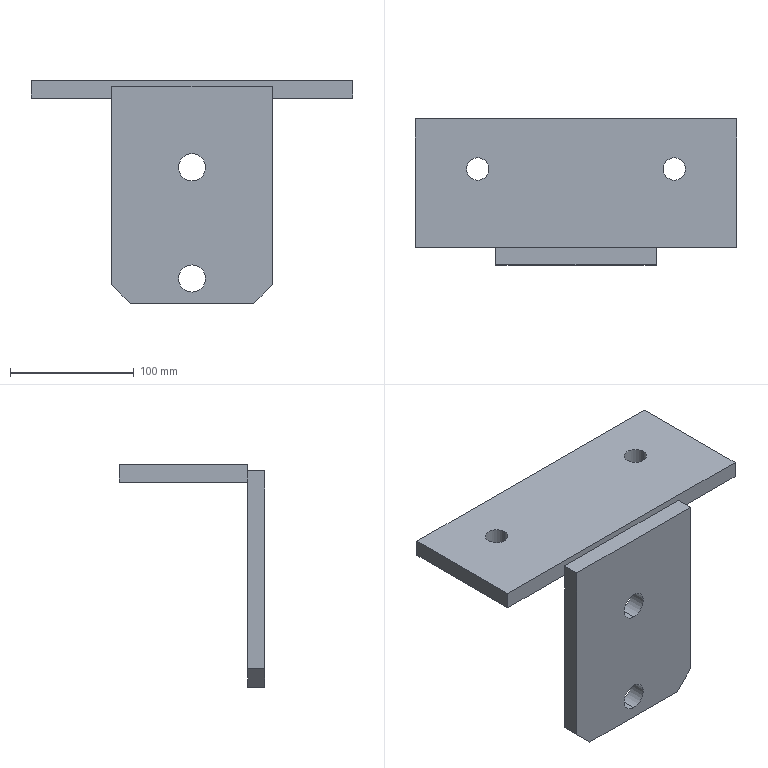Component | SolidWorks | LowerTensioningDeviceAssembly-1_GuideFrame-2 | 1 solid | 22 faces | box 260 x 117.9 x 180 mm | volume 675777 mm3 | plane 14 | cylinder 8 | commonest cylinder face diameters 18 x4 22 x4
build123d program:
from build123d import *

# Parameters (mm, degrees)
SKETCH1_W                 = 14
SKETCH1_H                 = 175
BOSS_EXTRUDE1_DEPTH       = 65
BOSS_EXTRUDE1_2_DEPTH     = 65
SKETCH2_W                 = 620
SKETCH2_H                 = 14
BOSS_EXTRUDE2_DEPTH       = 130
SKETCH3_R                 = 11
CUT_EXTRUDE1_DEPTH        = 685.985
CHAMFER1_SIZE             = 15
SKETCH4_W                 = 560.2
SKETCH4_H                 = 260
CUT_EXTRUDE2_DEPTH        = 393.78
SIZE_MM_DOWEL_PIN_HOLE1_D = 18


with BuildPart() as part:
    # Sketch1 → Boss-Extrude1 (new, symmetric)
    with BuildSketch(Plane.XY):
        with Locations((-317, 87.5)):
            Rectangle(SKETCH1_W, SKETCH1_H)
    extrude(amount=BOSS_EXTRUDE1_DEPTH, both=True)



with BuildPart() as body_2:
    # Sketch1 → Boss-Extrude1 2 (new, symmetric)
    with BuildSketch(Plane.XY):
        with Locations((317, 87.5)):
            Rectangle(SKETCH1_W, SKETCH1_H)
    extrude(amount=BOSS_EXTRUDE1_2_DEPTH, both=True)


with BuildPart() as part_1:
    add(part.part)

    add(body_2.part)  # Boss-Extrude2 merges body 2
    # Sketch2 → Boss-Extrude2 (add, symmetric)
    with BuildSketch(Plane.XY):
        with Locations((0, 173)):
            Rectangle(SKETCH2_W, SKETCH2_H)
    extrude(amount=BOSS_EXTRUDE2_DEPTH, both=True)

    # Sketch3 → Cut-Extrude1 (cut, through all)
    with BuildSketch(Plane(origin=(324, 0, 0), x_dir=(0, 0, -1), z_dir=(1, 0, 0))):
        with Locations(Location((0, 110, 0), (0, 0, 90))):
            Circle(SKETCH3_R)
        with Locations(Location((0, 20, 0), (0, 0, 90))):
            Circle(SKETCH3_R)
    extrude(amount=-CUT_EXTRUDE1_DEPTH, mode=Mode.SUBTRACT)

    # Chamfer1
    chamfer1_edges = [part_1.edges().sort_by_distance(p)[0] for p in [
        (317, 0, -65),
        (317, 0, 65),
        (-317, 0, -65),
        (-317, 0, 65),
    ]]
    chamfer(chamfer1_edges, length=CHAMFER1_SIZE)

    # Sketch4 → Cut-Extrude2 (cut, through all)
    with BuildSketch(Plane(origin=(0, 180, 0), x_dir=(1, 0, 0), z_dir=(0, 1, 0))):
        with Locations((74, 0)):
            Rectangle(SKETCH4_W, SKETCH4_H)
    extrude(amount=-CUT_EXTRUDE2_DEPTH, mode=Mode.SUBTRACT)

    # Size mm Dowel Pin Hole1 (through all)
    with Locations(Plane(origin=(0, 180, 0), x_dir=(1, 0, 0), z_dir=(0, 1, 0))):
        with Locations((-246.6, 79.5), (-246.6, -79.5)):
            Hole(SIZE_MM_DOWEL_PIN_HOLE1_D / 2)


solid = part_1.part

# Placed as in the assembly
solid = solid.moved(Location((0, -74, -270), (90, 90, 0)))
STEP:
#1=COLOUR_RGB('',0.7922,0.8196,0.9333);
#2=FILL_AREA_STYLE_COLOUR('',#1);
#3=FILL_AREA_STYLE('',(#2));
#4=SURFACE_STYLE_FILL_AREA(#3);
#5=SURFACE_SIDE_STYLE('',(#4));
#6=SURFACE_STYLE_USAGE(.BOTH.,#5);
#7=PRESENTATION_STYLE_ASSIGNMENT((#6));
#8=CARTESIAN_POINT('',(-3.484,-12.622,-4.094));
#9=VERTEX_POINT('',#8);
#10=CARTESIAN_POINT('',(-2.776,-12.622,-4.094));
#11=VERTEX_POINT('',#10);
#12=CARTESIAN_POINT('',(-3.13,-12.622,-4.094));
#13=DIRECTION('',(-0.,-0.,1.));
#14=DIRECTION('',(1.,0.,0.));
#15=AXIS2_PLACEMENT_3D('',#12,#13,#14);
#16=CIRCLE('',#15,0.3543);
#17=EDGE_CURVE('',#9,#11,#16,.T.);
#18=ORIENTED_EDGE('',*,*,#17,.F.);
#19=CARTESIAN_POINT('',(-3.484,-12.622,-3.543));
#20=VERTEX_POINT('',#19);
#21=CARTESIAN_POINT('',(-3.484,-12.622,-3.543));
#22=DIRECTION('',(-0.,-0.,1.));
#23=VECTOR('',#22,39.37);
#24=LINE('',#21,#23);
#25=EDGE_CURVE('',#9,#20,#24,.T.);
#26=ORIENTED_EDGE('',*,*,#25,.T.);
#27=CARTESIAN_POINT('',(-2.776,-12.622,-3.543));
#28=VERTEX_POINT('',#27);
#29=CARTESIAN_POINT('',(-3.13,-12.622,-3.543));
#30=DIRECTION('',(-0.,-0.,1.));
#31=DIRECTION('',(1.,0.,0.));
#32=AXIS2_PLACEMENT_3D('',#29,#30,#31);
#33=CIRCLE('',#32,0.3543);
#34=EDGE_CURVE('',#20,#28,#33,.T.);
#35=ORIENTED_EDGE('',*,*,#34,.T.);
#36=CARTESIAN_POINT('',(-2.776,-12.622,-3.543));
#37=DIRECTION('',(-0.,-0.,1.));
#38=VECTOR('',#37,39.37);
#39=LINE('',#36,#38);
#40=EDGE_CURVE('',#11,#28,#39,.T.);
#41=ORIENTED_EDGE('',*,*,#40,.F.);
#42=EDGE_LOOP('',(#18,#26,#35,#41));
#43=FACE_OUTER_BOUND('',#42,.T.);
#44=CARTESIAN_POINT('',(-3.13,-12.622,-3.543));
#45=DIRECTION('',(-0.,-0.,1.));
#46=DIRECTION('',(1.,0.,0.));
#47=AXIS2_PLACEMENT_3D('',#44,#45,#46);
#48=CYLINDRICAL_SURFACE('',#47,0.3543);
#49=ADVANCED_FACE('',(#43),#48,.F.);
#50=CARTESIAN_POINT('',(2.776,-12.622,-4.094));
#51=VERTEX_POINT('',#50);
#52=CARTESIAN_POINT('',(3.484,-12.622,-4.094));
#53=VERTEX_POINT('',#52);
#54=CARTESIAN_POINT('',(3.13,-12.622,-4.094));
#55=DIRECTION('',(-0.,-0.,1.));
#56=DIRECTION('',(1.,0.,0.));
#57=AXIS2_PLACEMENT_3D('',#54,#55,#56);
#58=CIRCLE('',#57,0.3543);
#59=EDGE_CURVE('',#51,#53,#58,.T.);
#60=ORIENTED_EDGE('',*,*,#59,.F.);
#61=CARTESIAN_POINT('',(2.776,-12.622,-3.543));
#62=VERTEX_POINT('',#61);
#63=CARTESIAN_POINT('',(2.776,-12.622,-3.543));
#64=DIRECTION('',(-0.,-0.,1.));
#65=VECTOR('',#64,39.37);
#66=LINE('',#63,#65);
#67=EDGE_CURVE('',#51,#62,#66,.T.);
#68=ORIENTED_EDGE('',*,*,#67,.T.);
#69=CARTESIAN_POINT('',(3.484,-12.622,-3.543));
#70=VERTEX_POINT('',#69);
#71=CARTESIAN_POINT('',(3.13,-12.622,-3.543));
#72=DIRECTION('',(-0.,-0.,1.));
#73=DIRECTION('',(1.,0.,0.));
#74=AXIS2_PLACEMENT_3D('',#71,#72,#73);
#75=CIRCLE('',#74,0.3543);
#76=EDGE_CURVE('',#62,#70,#75,.T.);
#77=ORIENTED_EDGE('',*,*,#76,.T.);
#78=CARTESIAN_POINT('',(3.484,-12.622,-3.543));
#79=DIRECTION('',(-0.,-0.,1.));
#80=VECTOR('',#79,39.37);
#81=LINE('',#78,#80);
#82=EDGE_CURVE('',#53,#70,#81,.T.);
#83=ORIENTED_EDGE('',*,*,#82,.F.);
#84=EDGE_LOOP('',(#60,#68,#77,#83));
#85=FACE_OUTER_BOUND('',#84,.T.);
#86=CARTESIAN_POINT('',(3.13,-12.622,-3.543));
#87=DIRECTION('',(-0.,-0.,1.));
#88=DIRECTION('',(1.,0.,0.));
#89=AXIS2_PLACEMENT_3D('',#86,#87,#88);
#90=CYLINDRICAL_SURFACE('',#89,0.3543);
#91=ADVANCED_FACE('',(#85),#90,.F.);
#92=CARTESIAN_POINT('',(-0.,-15.669,-10.276));
#93=VERTEX_POINT('',#92);
#94=CARTESIAN_POINT('',(-0.,-15.669,-9.409));
#95=VERTEX_POINT('',#94);
#96=CARTESIAN_POINT('',(-0.,-15.669,-9.843));
#97=DIRECTION('',(0.,1.,0.));
#98=DIRECTION('',(-0.,0.,1.));
#99=AXIS2_PLACEMENT_3D('',#96,#97,#98);
#100=CIRCLE('',#99,0.4331);
#101=EDGE_CURVE('',#93,#95,#100,.T.);
#102=ORIENTED_EDGE('',*,*,#101,.F.);
#103=CARTESIAN_POINT('',(-0.,-15.118,-10.276));
#104=VERTEX_POINT('',#103);
#105=CARTESIAN_POINT('',(-0.,-15.669,-10.276));
#106=DIRECTION('',(0.,1.,0.));
#107=VECTOR('',#106,39.37);
#108=LINE('',#105,#107);
#109=EDGE_CURVE('',#93,#104,#108,.T.);
#110=ORIENTED_EDGE('',*,*,#109,.T.);
#111=CARTESIAN_POINT('',(-0.,-15.118,-9.409));
#112=VERTEX_POINT('',#111);
#113=CARTESIAN_POINT('',(-0.,-15.118,-9.843));
#114=DIRECTION('',(-0.,-1.,-0.));
#115=DIRECTION('',(1.,0.,0.));
#116=AXIS2_PLACEMENT_3D('',#113,#114,#115);
#117=CIRCLE('',#116,0.4331);
#118=EDGE_CURVE('',#112,#104,#117,.T.);
#119=ORIENTED_EDGE('',*,*,#118,.F.);
#120=CARTESIAN_POINT('',(-0.,-15.669,-9.409));
#121=DIRECTION('',(0.,1.,0.));
#122=VECTOR('',#121,39.37);
#123=LINE('',#120,#122);
#124=EDGE_CURVE('',#95,#112,#123,.T.);
#125=ORIENTED_EDGE('',*,*,#124,.F.);
#126=EDGE_LOOP('',(#102,#110,#119,#125));
#127=FACE_OUTER_BOUND('',#126,.T.);
#128=CARTESIAN_POINT('',(-0.,-15.669,-9.843));
#129=DIRECTION('',(0.,1.,0.));
#130=DIRECTION('',(-0.,0.,1.));
#131=AXIS2_PLACEMENT_3D('',#128,#129,#130);
#132=CYLINDRICAL_SURFACE('',#131,0.4331);
#133=ADVANCED_FACE('',(#127),#132,.F.);
#134=CARTESIAN_POINT('',(-0.,-15.669,-6.732));
#135=VERTEX_POINT('',#134);
#136=CARTESIAN_POINT('',(-0.,-15.669,-5.866));
#137=VERTEX_POINT('',#136);
#138=CARTESIAN_POINT('',(-0.,-15.669,-6.299));
#139=DIRECTION('',(0.,1.,0.));
#140=DIRECTION('',(-0.,0.,1.));
#141=AXIS2_PLACEMENT_3D('',#138,#139,#140);
#142=CIRCLE('',#141,0.4331);
#143=EDGE_CURVE('',#135,#137,#142,.T.);
#144=ORIENTED_EDGE('',*,*,#143,.F.);
#145=CARTESIAN_POINT('',(-0.,-15.118,-6.732));
#146=VERTEX_POINT('',#145);
#147=CARTESIAN_POINT('',(-0.,-15.669,-6.732));
#148=DIRECTION('',(0.,1.,0.));
#149=VECTOR('',#148,39.37);
#150=LINE('',#147,#149);
#151=EDGE_CURVE('',#135,#146,#150,.T.);
#152=ORIENTED_EDGE('',*,*,#151,.T.);
#153=CARTESIAN_POINT('',(-0.,-15.118,-5.866));
#154=VERTEX_POINT('',#153);
#155=CARTESIAN_POINT('',(-0.,-15.118,-6.299));
#156=DIRECTION('',(-0.,-1.,-0.));
#157=DIRECTION('',(1.,0.,0.));
#158=AXIS2_PLACEMENT_3D('',#155,#156,#157);
#159=CIRCLE('',#158,0.4331);
#160=EDGE_CURVE('',#154,#146,#159,.T.);
#161=ORIENTED_EDGE('',*,*,#160,.F.);
#162=CARTESIAN_POINT('',(-0.,-15.669,-5.866));
#163=DIRECTION('',(0.,1.,0.));
#164=VECTOR('',#163,39.37);
#165=LINE('',#162,#164);
#166=EDGE_CURVE('',#137,#154,#165,.T.);
#167=ORIENTED_EDGE('',*,*,#166,.F.);
#168=EDGE_LOOP('',(#144,#152,#161,#167));
#169=FACE_OUTER_BOUND('',#168,.T.);
#170=CARTESIAN_POINT('',(-0.,-15.669,-6.299));
#171=DIRECTION('',(0.,1.,0.));
#172=DIRECTION('',(-0.,0.,1.));
#173=AXIS2_PLACEMENT_3D('',#170,#171,#172);
#174=CYLINDRICAL_SURFACE('',#173,0.4331);
#175=ADVANCED_FACE('',(#169),#174,.F.);
#176=ORIENTED_EDGE('',*,*,#118,.T.);
#177=CARTESIAN_POINT('',(-0.,-15.118,-9.843));
#178=DIRECTION('',(-0.,-1.,-0.));
#179=DIRECTION('',(1.,0.,0.));
#180=AXIS2_PLACEMENT_3D('',#177,#178,#179);
#181=CIRCLE('',#180,0.4331);
#182=EDGE_CURVE('',#104,#112,#181,.T.);
#183=ORIENTED_EDGE('',*,*,#182,.T.);
#184=EDGE_LOOP('',(#176,#183));
#185=FACE_BOUND('',#184,.T.);
#186=ORIENTED_EDGE('',*,*,#160,.T.);
#187=CARTESIAN_POINT('',(-0.,-15.118,-6.299));
#188=DIRECTION('',(-0.,-1.,-0.));
#189=DIRECTION('',(1.,0.,0.));
#190=AXIS2_PLACEMENT_3D('',#187,#188,#189);
#191=CIRCLE('',#190,0.4331);
#192=EDGE_CURVE('',#146,#154,#191,.T.);
#193=ORIENTED_EDGE('',*,*,#192,.T.);
#194=EDGE_LOOP('',(#186,#193));
#195=FACE_BOUND('',#194,.T.);
#196=CARTESIAN_POINT('',(1.969,-15.118,-10.63));
#197=VERTEX_POINT('',#196);
#198=CARTESIAN_POINT('',(-1.969,-15.118,-10.63));
#199=VERTEX_POINT('',#198);
#200=CARTESIAN_POINT('',(2.559,-15.118,-10.63));
#201=DIRECTION('',(-1.,0.,-0.));
#202=VECTOR('',#201,39.37);
#203=LINE('',#200,#202);
#204=EDGE_CURVE('',#197,#199,#203,.T.);
#205=ORIENTED_EDGE('',*,*,#204,.T.);
#206=CARTESIAN_POINT('',(-2.559,-15.118,-10.039));
#207=VERTEX_POINT('',#206);
#208=CARTESIAN_POINT('',(-1.969,-15.118,-10.63));
#209=DIRECTION('',(-0.7071,-0.,0.7071));
#210=VECTOR('',#209,39.37);
#211=LINE('',#208,#210);
#212=EDGE_CURVE('',#199,#207,#211,.T.);
#213=ORIENTED_EDGE('',*,*,#212,.T.);
#214=CARTESIAN_POINT('',(-2.559,-15.118,-4.094));
#215=VERTEX_POINT('',#214);
#216=CARTESIAN_POINT('',(-2.559,-15.118,-3.74));
#217=DIRECTION('',(-0.,-0.,1.));
#218=VECTOR('',#217,39.37);
#219=LINE('',#216,#218);
#220=EDGE_CURVE('',#207,#215,#219,.T.);
#221=ORIENTED_EDGE('',*,*,#220,.T.);
#222=CARTESIAN_POINT('',(2.559,-15.118,-4.094));
#223=VERTEX_POINT('',#222);
#224=CARTESIAN_POINT('',(5.118,-15.118,-4.094));
#225=DIRECTION('',(-1.,0.,-0.));
#226=VECTOR('',#225,39.37);
#227=LINE('',#224,#226);
#228=EDGE_CURVE('',#223,#215,#227,.T.);
#229=ORIENTED_EDGE('',*,*,#228,.F.);
#230=CARTESIAN_POINT('',(2.559,-15.118,-10.039));
#231=VERTEX_POINT('',#230);
#232=CARTESIAN_POINT('',(2.559,-15.118,-3.74));
#233=DIRECTION('',(-0.,-0.,1.));
#234=VECTOR('',#233,39.37);
#235=LINE('',#232,#234);
#236=EDGE_CURVE('',#231,#223,#235,.T.);
#237=ORIENTED_EDGE('',*,*,#236,.F.);
#238=CARTESIAN_POINT('',(2.559,-15.118,-10.039));
#239=DIRECTION('',(-0.7071,0.,-0.7071));
#240=VECTOR('',#239,39.37);
#241=LINE('',#238,#240);
#242=EDGE_CURVE('',#231,#197,#241,.T.);
#243=ORIENTED_EDGE('',*,*,#242,.T.);
#244=EDGE_LOOP('',(#205,#213,#221,#229,#237,#243));
#245=FACE_OUTER_BOUND('',#244,.T.);
#246=CARTESIAN_POINT('',(2.559,-15.118,-3.74));
#247=DIRECTION('',(-0.,-1.,-0.));
#248=DIRECTION('',(1.,-0.,0.));
#249=AXIS2_PLACEMENT_3D('',#246,#247,#248);
#250=PLANE('',#249);
#251=ADVANCED_FACE('',(#185,#195,#245),#250,.F.);
#252=CARTESIAN_POINT('',(-0.,-15.669,-9.843));
#253=DIRECTION('',(0.,1.,0.));
#254=DIRECTION('',(-0.,0.,1.));
#255=AXIS2_PLACEMENT_3D('',#252,#253,#254);
#256=CIRCLE('',#255,0.4331);
#257=EDGE_CURVE('',#95,#93,#256,.T.);
#258=ORIENTED_EDGE('',*,*,#257,.T.);
#259=ORIENTED_EDGE('',*,*,#101,.T.);
#260=EDGE_LOOP('',(#258,#259));
#261=FACE_BOUND('',#260,.T.);
#262=CARTESIAN_POINT('',(-0.,-15.669,-6.299));
#263=DIRECTION('',(0.,1.,0.));
#264=DIRECTION('',(-0.,0.,1.));
#265=AXIS2_PLACEMENT_3D('',#262,#263,#264);
#266=CIRCLE('',#265,0.4331);
#267=EDGE_CURVE('',#137,#135,#266,.T.);
#268=ORIENTED_EDGE('',*,*,#267,.T.);
#269=ORIENTED_EDGE('',*,*,#143,.T.);
#270=EDGE_LOOP('',(#268,#269));
#271=FACE_BOUND('',#270,.T.);
#272=CARTESIAN_POINT('',(-2.559,-15.669,-3.74));
#273=VERTEX_POINT('',#272);
#274=CARTESIAN_POINT('',(-2.559,-15.669,-10.039));
#275=VERTEX_POINT('',#274);
#276=CARTESIAN_POINT('',(-2.559,-15.669,-3.74));
#277=DIRECTION('',(0.,0.,-1.));
#278=VECTOR('',#277,39.37);
#279=LINE('',#276,#278);
#280=EDGE_CURVE('',#273,#275,#279,.T.);
#281=ORIENTED_EDGE('',*,*,#280,.T.);
#282=CARTESIAN_POINT('',(-1.969,-15.669,-10.63));
#283=VERTEX_POINT('',#282);
#284=CARTESIAN_POINT('',(-1.969,-15.669,-10.63));
#285=DIRECTION('',(0.7071,0.,-0.7071));
#286=VECTOR('',#285,39.37);
#287=LINE('',#284,#286);
#288=EDGE_CURVE('',#275,#283,#287,.T.);
#289=ORIENTED_EDGE('',*,*,#288,.T.);
#290=CARTESIAN_POINT('',(1.969,-15.669,-10.63));
#291=VERTEX_POINT('',#290);
#292=CARTESIAN_POINT('',(2.559,-15.669,-10.63));
#293=DIRECTION('',(-1.,0.,-0.));
#294=VECTOR('',#293,39.37);
#295=LINE('',#292,#294);
#296=EDGE_CURVE('',#291,#283,#295,.T.);
#297=ORIENTED_EDGE('',*,*,#296,.F.);
#298=CARTESIAN_POINT('',(2.559,-15.669,-10.039));
#299=VERTEX_POINT('',#298);
#300=CARTESIAN_POINT('',(2.559,-15.669,-10.039));
#301=DIRECTION('',(0.7071,-0.,0.7071));
#302=VECTOR('',#301,39.37);
#303=LINE('',#300,#302);
#304=EDGE_CURVE('',#291,#299,#303,.T.);
#305=ORIENTED_EDGE('',*,*,#304,.T.);
#306=CARTESIAN_POINT('',(2.559,-15.669,-3.74));
#307=VERTEX_POINT('',#306);
#308=CARTESIAN_POINT('',(2.559,-15.669,-3.74));
#309=DIRECTION('',(0.,0.,-1.));
#310=VECTOR('',#309,39.37);
#311=LINE('',#308,#310);
#312=EDGE_CURVE('',#307,#299,#311,.T.);
#313=ORIENTED_EDGE('',*,*,#312,.F.);
#314=CARTESIAN_POINT('',(2.559,-15.669,-3.74));
#315=DIRECTION('',(-1.,0.,-0.));
#316=VECTOR('',#315,39.37);
#317=LINE('',#314,#316);
#318=EDGE_CURVE('',#307,#273,#317,.T.);
#319=ORIENTED_EDGE('',*,*,#318,.T.);
#320=EDGE_LOOP('',(#281,#289,#297,#305,#313,#319));
#321=FACE_OUTER_BOUND('',#320,.T.);
#322=CARTESIAN_POINT('',(2.559,-15.669,-3.74));
#323=DIRECTION('',(0.,1.,0.));
#324=DIRECTION('',(-0.,-0.,1.));
#325=AXIS2_PLACEMENT_3D('',#322,#323,#324);
#326=PLANE('',#325);
#327=ADVANCED_FACE('',(#261,#271,#321),#326,.F.);
#328=ORIENTED_EDGE('',*,*,#296,.T.);
#329=CARTESIAN_POINT('',(-1.969,-15.669,-10.63));
#330=DIRECTION('',(0.,1.,0.));
#331=VECTOR('',#330,39.37);
#332=LINE('',#329,#331);
#333=EDGE_CURVE('',#283,#199,#332,.T.);
#334=ORIENTED_EDGE('',*,*,#333,.T.);
#335=ORIENTED_EDGE('',*,*,#204,.F.);
#336=CARTESIAN_POINT('',(1.969,-15.669,-10.63));
#337=DIRECTION('',(-0.,-1.,-0.));
#338=VECTOR('',#337,39.37);
#339=LINE('',#336,#338);
#340=EDGE_CURVE('',#197,#291,#339,.T.);
#341=ORIENTED_EDGE('',*,*,#340,.T.);
#342=EDGE_LOOP('',(#328,#334,#335,#341));
#343=FACE_OUTER_BOUND('',#342,.T.);
#344=CARTESIAN_POINT('',(2.559,-15.669,-10.63));
#345=DIRECTION('',(-0.,-0.,1.));
#346=DIRECTION('',(1.,-0.,0.));
#347=AXIS2_PLACEMENT_3D('',#344,#345,#346);
#348=PLANE('',#347);
#349=ADVANCED_FACE('',(#343),#348,.F.);
#350=CARTESIAN_POINT('',(-2.559,-15.118,-3.74));
#351=VERTEX_POINT('',#350);
#352=CARTESIAN_POINT('',(-2.559,-15.669,-3.74));
#353=DIRECTION('',(-0.,-1.,-0.));
#354=VECTOR('',#353,39.37);
#355=LINE('',#352,#354);
#356=EDGE_CURVE('',#351,#273,#355,.T.);
#357=ORIENTED_EDGE('',*,*,#356,.T.);
#358=ORIENTED_EDGE('',*,*,#318,.F.);
#359=CARTESIAN_POINT('',(2.559,-15.118,-3.74));
#360=VERTEX_POINT('',#359);
#361=CARTESIAN_POINT('',(2.559,-15.669,-3.74));
#362=DIRECTION('',(-0.,-1.,-0.));
#363=VECTOR('',#362,39.37);
#364=LINE('',#361,#363);
#365=EDGE_CURVE('',#360,#307,#364,.T.);
#366=ORIENTED_EDGE('',*,*,#365,.F.);
#367=CARTESIAN_POINT('',(2.559,-15.118,-3.74));
#368=DIRECTION('',(-1.,0.,-0.));
#369=VECTOR('',#368,39.37);
#370=LINE('',#367,#369);
#371=EDGE_CURVE('',#360,#351,#370,.T.);
#372=ORIENTED_EDGE('',*,*,#371,.T.);
#373=EDGE_LOOP('',(#357,#358,#366,#372));
#374=FACE_OUTER_BOUND('',#373,.T.);
#375=CARTESIAN_POINT('',(2.559,-15.669,-3.74));
#376=DIRECTION('',(0.,0.,-1.));
#377=DIRECTION('',(-1.,0.,-0.));
#378=AXIS2_PLACEMENT_3D('',#375,#376,#377);
#379=PLANE('',#378);
#380=ADVANCED_FACE('',(#374),#379,.F.);
#381=ORIENTED_EDGE('',*,*,#312,.T.);
#382=CARTESIAN_POINT('',(2.559,-15.118,-10.039));
#383=DIRECTION('',(0.,1.,0.));
#384=VECTOR('',#383,39.37);
#385=LINE('',#382,#384);
#386=EDGE_CURVE('',#299,#231,#385,.T.);
#387=ORIENTED_EDGE('',*,*,#386,.T.);
#388=ORIENTED_EDGE('',*,*,#236,.T.);
#389=CARTESIAN_POINT('',(2.559,-15.118,-3.74));
#390=DIRECTION('',(-0.,-0.,1.));
#391=VECTOR('',#390,39.37);
#392=LINE('',#389,#391);
#393=EDGE_CURVE('',#223,#360,#392,.T.);
#394=ORIENTED_EDGE('',*,*,#393,.T.);
#395=ORIENTED_EDGE('',*,*,#365,.T.);
#396=EDGE_LOOP('',(#381,#387,#388,#394,#395));
#397=FACE_OUTER_BOUND('',#396,.T.);
#398=CARTESIAN_POINT('',(2.559,-2.913,-10.63));
#399=DIRECTION('',(1.,-0.,0.));
#400=DIRECTION('',(0.,1.,0.));
#401=AXIS2_PLACEMENT_3D('',#398,#399,#400);
#402=PLANE('',#401);
#403=ADVANCED_FACE('',(#397),#402,.T.);
#404=ORIENTED_EDGE('',*,*,#220,.F.);
#405=CARTESIAN_POINT('',(-2.559,-2.913,-10.039));
#406=DIRECTION('',(-0.,-1.,-0.));
#407=VECTOR('',#406,39.37);
#408=LINE('',#405,#407);
#409=EDGE_CURVE('',#207,#275,#408,.T.);
#410=ORIENTED_EDGE('',*,*,#409,.T.);
#411=ORIENTED_EDGE('',*,*,#280,.F.);
#412=ORIENTED_EDGE('',*,*,#356,.F.);
#413=CARTESIAN_POINT('',(-2.559,-15.118,-3.74));
#414=DIRECTION('',(-0.,-0.,1.));
#415=VECTOR('',#414,39.37);
#416=LINE('',#413,#415);
#417=EDGE_CURVE('',#215,#351,#416,.T.);
#418=ORIENTED_EDGE('',*,*,#417,.F.);
#419=EDGE_LOOP('',(#404,#410,#411,#412,#418));
#420=FACE_OUTER_BOUND('',#419,.T.);
#421=CARTESIAN_POINT('',(-2.559,-2.913,-10.63));
#422=DIRECTION('',(1.,-0.,0.));
#423=DIRECTION('',(0.,1.,0.));
#424=AXIS2_PLACEMENT_3D('',#421,#422,#423);
#425=PLANE('',#424);
#426=ADVANCED_FACE('',(#420),#425,.F.);
#427=CARTESIAN_POINT('',(-5.118,-15.118,-4.094));
#428=VERTEX_POINT('',#427);
#429=CARTESIAN_POINT('',(5.118,-15.118,-4.094));
#430=DIRECTION('',(-1.,0.,-0.));
#431=VECTOR('',#430,39.37);
#432=LINE('',#429,#431);
#433=EDGE_CURVE('',#215,#428,#432,.T.);
#434=ORIENTED_EDGE('',*,*,#433,.F.);
#435=ORIENTED_EDGE('',*,*,#417,.T.);
#436=ORIENTED_EDGE('',*,*,#371,.F.);
#437=ORIENTED_EDGE('',*,*,#393,.F.);
#438=CARTESIAN_POINT('',(5.118,-15.118,-4.094));
#439=VERTEX_POINT('',#438);
#440=CARTESIAN_POINT('',(5.118,-15.118,-4.094));
#441=DIRECTION('',(-1.,0.,-0.));
#442=VECTOR('',#441,39.37);
#443=LINE('',#440,#442);
#444=EDGE_CURVE('',#439,#223,#443,.T.);
#445=ORIENTED_EDGE('',*,*,#444,.F.);
#446=CARTESIAN_POINT('',(5.118,-15.118,-3.543));
#447=VERTEX_POINT('',#446);
#448=CARTESIAN_POINT('',(5.118,-15.118,-4.094));
#449=DIRECTION('',(0.,0.,-1.));
#450=VECTOR('',#449,39.37);
#451=LINE('',#448,#450);
#452=EDGE_CURVE('',#447,#439,#451,.T.);
#453=ORIENTED_EDGE('',*,*,#452,.F.);
#454=CARTESIAN_POINT('',(-5.118,-15.118,-3.543));
#455=VERTEX_POINT('',#454);
#456=CARTESIAN_POINT('',(5.118,-15.118,-3.543));
#457=DIRECTION('',(-1.,0.,-0.));
#458=VECTOR('',#457,39.37);
#459=LINE('',#456,#458);
#460=EDGE_CURVE('',#447,#455,#459,.T.);
#461=ORIENTED_EDGE('',*,*,#460,.T.);
#462=CARTESIAN_POINT('',(-5.118,-15.118,-4.094));
#463=DIRECTION('',(0.,0.,-1.));
#464=VECTOR('',#463,39.37);
#465=LINE('',#462,#464);
#466=EDGE_CURVE('',#455,#428,#465,.T.);
#467=ORIENTED_EDGE('',*,*,#466,.T.);
#468=EDGE_LOOP('',(#434,#435,#436,#437,#445,#453,#461,#467));
#469=FACE_OUTER_BOUND('',#468,.T.);
#470=CARTESIAN_POINT('',(5.118,-15.118,-4.094));
#471=DIRECTION('',(0.,1.,0.));
#472=DIRECTION('',(-1.,0.,-0.));
#473=AXIS2_PLACEMENT_3D('',#470,#471,#472);
#474=PLANE('',#473);
#475=ADVANCED_FACE('',(#469),#474,.F.);
#476=CARTESIAN_POINT('',(-3.13,-12.622,-4.094));
#477=DIRECTION('',(-0.,-0.,1.));
#478=DIRECTION('',(1.,0.,0.));
#479=AXIS2_PLACEMENT_3D('',#476,#477,#478);
#480=CIRCLE('',#479,0.3543);
#481=EDGE_CURVE('',#11,#9,#480,.T.);
#482=ORIENTED_EDGE('',*,*,#481,.T.);
#483=ORIENTED_EDGE('',*,*,#17,.T.);
#484=EDGE_LOOP('',(#482,#483));
#485=FACE_BOUND('',#484,.T.);
#486=CARTESIAN_POINT('',(3.13,-12.622,-4.094));
#487=DIRECTION('',(-0.,-0.,1.));
#488=DIRECTION('',(1.,0.,0.));
#489=AXIS2_PLACEMENT_3D('',#486,#487,#488);
#490=CIRCLE('',#489,0.3543);
#491=EDGE_CURVE('',#53,#51,#490,.T.);
#492=ORIENTED_EDGE('',*,*,#491,.T.);
#493=ORIENTED_EDGE('',*,*,#59,.T.);
#494=EDGE_LOOP('',(#492,#493));
#495=FACE_BOUND('',#494,.T.);
#496=CARTESIAN_POINT('',(-5.118,-11.028,-4.094));
#497=VERTEX_POINT('',#496);
#498=CARTESIAN_POINT('',(-5.118,-15.118,-4.094));
#499=DIRECTION('',(0.,1.,0.));
#500=VECTOR('',#499,39.37);
#501=LINE('',#498,#500);
#502=EDGE_CURVE('',#428,#497,#501,.T.);
#503=ORIENTED_EDGE('',*,*,#502,.T.);
#504=CARTESIAN_POINT('',(5.118,-11.028,-4.094));
#505=VERTEX_POINT('',#504);
#506=CARTESIAN_POINT('',(5.118,-11.028,-4.094));
#507=DIRECTION('',(1.,-0.,0.));
#508=VECTOR('',#507,39.37);
#509=LINE('',#506,#508);
#510=EDGE_CURVE('',#497,#505,#509,.T.);
#511=ORIENTED_EDGE('',*,*,#510,.T.);
#512=CARTESIAN_POINT('',(5.118,-15.118,-4.094));
#513=DIRECTION('',(0.,1.,0.));
#514=VECTOR('',#513,39.37);
#515=LINE('',#512,#514);
#516=EDGE_CURVE('',#439,#505,#515,.T.);
#517=ORIENTED_EDGE('',*,*,#516,.F.);
#518=ORIENTED_EDGE('',*,*,#444,.T.);
#519=ORIENTED_EDGE('',*,*,#228,.T.);
#520=ORIENTED_EDGE('',*,*,#433,.T.);
#521=EDGE_LOOP('',(#503,#511,#517,#518,#519,#520));
#522=FACE_OUTER_BOUND('',#521,.T.);
#523=CARTESIAN_POINT('',(5.118,-15.118,-4.094));
#524=DIRECTION('',(-0.,-0.,1.));
#525=DIRECTION('',(1.,-0.,0.));
#526=AXIS2_PLACEMENT_3D('',#523,#524,#525);
#527=PLANE('',#526);
#528=ADVANCED_FACE('',(#485,#495,#522),#527,.F.);
#529=CARTESIAN_POINT('',(-3.13,-12.622,-3.543));
#530=DIRECTION('',(-0.,-0.,1.));
#531=DIRECTION('',(1.,0.,0.));
#532=AXIS2_PLACEMENT_3D('',#529,#530,#531);
#533=CIRCLE('',#532,0.3543);
#534=EDGE_CURVE('',#28,#20,#533,.T.);
#535=ORIENTED_EDGE('',*,*,#534,.F.);
#536=ORIENTED_EDGE('',*,*,#34,.F.);
#537=EDGE_LOOP('',(#535,#536));
#538=FACE_BOUND('',#537,.T.);
#539=CARTESIAN_POINT('',(3.13,-12.622,-3.543));
#540=DIRECTION('',(-0.,-0.,1.));
#541=DIRECTION('',(1.,0.,0.));
#542=AXIS2_PLACEMENT_3D('',#539,#540,#541);
#543=CIRCLE('',#542,0.3543);
#544=EDGE_CURVE('',#70,#62,#543,.T.);
#545=ORIENTED_EDGE('',*,*,#544,.F.);
#546=ORIENTED_EDGE('',*,*,#76,.F.);
#547=EDGE_LOOP('',(#545,#546));
#548=FACE_BOUND('',#547,.T.);
#549=CARTESIAN_POINT('',(5.118,-11.028,-3.543));
#550=VERTEX_POINT('',#549);
#551=CARTESIAN_POINT('',(5.118,-15.118,-3.543));
#552=DIRECTION('',(-0.,-1.,-0.));
#553=VECTOR('',#552,39.37);
#554=LINE('',#551,#553);
#555=EDGE_CURVE('',#550,#447,#554,.T.);
#556=ORIENTED_EDGE('',*,*,#555,.F.);
#557=CARTESIAN_POINT('',(-5.118,-11.028,-3.543));
#558=VERTEX_POINT('',#557);
#559=CARTESIAN_POINT('',(-5.118,-11.028,-3.543));
#560=DIRECTION('',(1.,-0.,0.));
#561=VECTOR('',#560,39.37);
#562=LINE('',#559,#561);
#563=EDGE_CURVE('',#558,#550,#562,.T.);
#564=ORIENTED_EDGE('',*,*,#563,.F.);
#565=CARTESIAN_POINT('',(-5.118,-15.118,-3.543));
#566=DIRECTION('',(-0.,-1.,-0.));
#567=VECTOR('',#566,39.37);
#568=LINE('',#565,#567);
#569=EDGE_CURVE('',#558,#455,#568,.T.);
#570=ORIENTED_EDGE('',*,*,#569,.T.);
#571=ORIENTED_EDGE('',*,*,#460,.F.);
#572=EDGE_LOOP('',(#556,#564,#570,#571));
#573=FACE_OUTER_BOUND('',#572,.T.);
#574=CARTESIAN_POINT('',(5.118,-15.118,-3.543));
#575=DIRECTION('',(0.,0.,-1.));
#576=DIRECTION('',(-1.,0.,-0.));
#577=AXIS2_PLACEMENT_3D('',#574,#575,#576);
#578=PLANE('',#577);
#579=ADVANCED_FACE('',(#538,#548,#573),#578,.F.);
#580=ORIENTED_EDGE('',*,*,#516,.T.);
#581=CARTESIAN_POINT('',(5.118,-11.028,-10.63));
#582=DIRECTION('',(-0.,-0.,1.));
#583=VECTOR('',#582,39.37);
#584=LINE('',#581,#583);
#585=EDGE_CURVE('',#505,#550,#584,.T.);
#586=ORIENTED_EDGE('',*,*,#585,.T.);
#587=ORIENTED_EDGE('',*,*,#555,.T.);
#588=ORIENTED_EDGE('',*,*,#452,.T.);
#589=EDGE_LOOP('',(#580,#586,#587,#588));
#590=FACE_OUTER_BOUND('',#589,.T.);
#591=CARTESIAN_POINT('',(5.118,-2.913,-10.63));
#592=DIRECTION('',(-1.,0.,-0.));
#593=DIRECTION('',(-0.,-1.,-0.));
#594=AXIS2_PLACEMENT_3D('',#591,#592,#593);
#595=PLANE('',#594);
#596=ADVANCED_FACE('',(#590),#595,.F.);
#597=CARTESIAN_POINT('',(-5.118,-11.028,-10.63));
#598=DIRECTION('',(-0.,-0.,1.));
#599=VECTOR('',#598,39.37);
#600=LINE('',#597,#599);
#601=EDGE_CURVE('',#497,#558,#600,.T.);
#602=ORIENTED_EDGE('',*,*,#601,.F.);
#603=ORIENTED_EDGE('',*,*,#502,.F.);
#604=ORIENTED_EDGE('',*,*,#466,.F.);
#605=ORIENTED_EDGE('',*,*,#569,.F.);
#606=EDGE_LOOP('',(#602,#603,#604,#605));
#607=FACE_OUTER_BOUND('',#606,.T.);
#608=CARTESIAN_POINT('',(-5.118,-2.913,-10.63));
#609=DIRECTION('',(-1.,0.,-0.));
#610=DIRECTION('',(-0.,-1.,-0.));
#611=AXIS2_PLACEMENT_3D('',#608,#609,#610);
#612=PLANE('',#611);
#613=ADVANCED_FACE('',(#607),#612,.T.);
#614=ORIENTED_EDGE('',*,*,#151,.F.);
#615=ORIENTED_EDGE('',*,*,#267,.F.);
#616=ORIENTED_EDGE('',*,*,#166,.T.);
#617=ORIENTED_EDGE('',*,*,#192,.F.);
#618=EDGE_LOOP('',(#614,#615,#616,#617));
#619=FACE_OUTER_BOUND('',#618,.T.);
#620=CARTESIAN_POINT('',(-0.,-15.669,-6.299));
#621=DIRECTION('',(0.,1.,0.));
#622=DIRECTION('',(-0.,0.,1.));
#623=AXIS2_PLACEMENT_3D('',#620,#621,#622);
#624=CYLINDRICAL_SURFACE('',#623,0.4331);
#625=ADVANCED_FACE('',(#619),#624,.F.);
#626=ORIENTED_EDGE('',*,*,#109,.F.);
#627=ORIENTED_EDGE('',*,*,#257,.F.);
#628=ORIENTED_EDGE('',*,*,#124,.T.);
#629=ORIENTED_EDGE('',*,*,#182,.F.);
#630=EDGE_LOOP('',(#626,#627,#628,#629));
#631=FACE_OUTER_BOUND('',#630,.T.);
#632=CARTESIAN_POINT('',(-0.,-15.669,-9.843));
#633=DIRECTION('',(0.,1.,0.));
#634=DIRECTION('',(-0.,0.,1.));
#635=AXIS2_PLACEMENT_3D('',#632,#633,#634);
#636=CYLINDRICAL_SURFACE('',#635,0.4331);
#637=ADVANCED_FACE('',(#631),#636,.F.);
#638=ORIENTED_EDGE('',*,*,#288,.F.);
#639=ORIENTED_EDGE('',*,*,#409,.F.);
#640=ORIENTED_EDGE('',*,*,#212,.F.);
#641=ORIENTED_EDGE('',*,*,#333,.F.);
#642=EDGE_LOOP('',(#638,#639,#640,#641));
#643=FACE_OUTER_BOUND('',#642,.T.);
#644=CARTESIAN_POINT('',(-1.969,-15.669,-10.63));
#645=DIRECTION('',(0.7071,-0.,0.7071));
#646=DIRECTION('',(0.,1.,0.));
#647=AXIS2_PLACEMENT_3D('',#644,#645,#646);
#648=PLANE('',#647);
#649=ADVANCED_FACE('',(#643),#648,.F.);
#650=ORIENTED_EDGE('',*,*,#304,.F.);
#651=ORIENTED_EDGE('',*,*,#340,.F.);
#652=ORIENTED_EDGE('',*,*,#242,.F.);
#653=ORIENTED_EDGE('',*,*,#386,.F.);
#654=EDGE_LOOP('',(#650,#651,#652,#653));
#655=FACE_OUTER_BOUND('',#654,.T.);
#656=CARTESIAN_POINT('',(2.559,-2.913,-10.039));
#657=DIRECTION('',(0.7071,0.,-0.7071));
#658=DIRECTION('',(-0.,-1.,-0.));
#659=AXIS2_PLACEMENT_3D('',#656,#657,#658);
#660=PLANE('',#659);
#661=ADVANCED_FACE('',(#655),#660,.T.);
#662=ORIENTED_EDGE('',*,*,#601,.T.);
#663=ORIENTED_EDGE('',*,*,#563,.T.);
#664=ORIENTED_EDGE('',*,*,#585,.F.);
#665=ORIENTED_EDGE('',*,*,#510,.F.);
#666=EDGE_LOOP('',(#662,#663,#664,#665));
#667=FACE_OUTER_BOUND('',#666,.T.);
#668=CARTESIAN_POINT('',(-5.118,-11.028,-10.63));
#669=DIRECTION('',(-0.,-1.,-0.));
#670=DIRECTION('',(1.,-0.,0.));
#671=AXIS2_PLACEMENT_3D('',#668,#669,#670);
#672=PLANE('',#671);
#673=ADVANCED_FACE('',(#667),#672,.F.);
#674=ORIENTED_EDGE('',*,*,#67,.F.);
#675=ORIENTED_EDGE('',*,*,#491,.F.);
#676=ORIENTED_EDGE('',*,*,#82,.T.);
#677=ORIENTED_EDGE('',*,*,#544,.T.);
#678=EDGE_LOOP('',(#674,#675,#676,#677));
#679=FACE_OUTER_BOUND('',#678,.T.);
#680=CARTESIAN_POINT('',(3.13,-12.622,-3.543));
#681=DIRECTION('',(-0.,-0.,1.));
#682=DIRECTION('',(1.,0.,0.));
#683=AXIS2_PLACEMENT_3D('',#680,#681,#682);
#684=CYLINDRICAL_SURFACE('',#683,0.3543);
#685=ADVANCED_FACE('',(#679),#684,.F.);
#686=ORIENTED_EDGE('',*,*,#25,.F.);
#687=ORIENTED_EDGE('',*,*,#481,.F.);
#688=ORIENTED_EDGE('',*,*,#40,.T.);
#689=ORIENTED_EDGE('',*,*,#534,.T.);
#690=EDGE_LOOP('',(#686,#687,#688,#689));
#691=FACE_OUTER_BOUND('',#690,.T.);
#692=CARTESIAN_POINT('',(-3.13,-12.622,-3.543));
#693=DIRECTION('',(-0.,-0.,1.));
#694=DIRECTION('',(1.,0.,0.));
#695=AXIS2_PLACEMENT_3D('',#692,#693,#694);
#696=CYLINDRICAL_SURFACE('',#695,0.3543);
#697=ADVANCED_FACE('',(#691),#696,.F.);
#698=CLOSED_SHELL('',(#49,#91,#133,#175,#251,#327,#349,#380,#403,#426,#475,#528,#579,#596,#613,#625,#637,#649,#661,#673,#685,#697));
#699=MANIFOLD_SOLID_BREP('',#698);
#700=STYLED_ITEM('',(#7),#699);
#701=(LENGTH_UNIT()NAMED_UNIT(*)SI_UNIT($,.METRE.));
#702=LENGTH_MEASURE_WITH_UNIT(LENGTH_MEASURE(0.0254),#701);
#703=DIMENSIONAL_EXPONENTS(1.,0.,0.,0.,0.,0.,0.);
#704=(CONVERSION_BASED_UNIT('',#702)LENGTH_UNIT()NAMED_UNIT(#703));
#705=UNCERTAINTY_MEASURE_WITH_UNIT(LENGTH_MEASURE(0.00001),#704,'','');
#706=(NAMED_UNIT(*)PLANE_ANGLE_UNIT()SI_UNIT($,.RADIAN.));
#707=(NAMED_UNIT(*)SI_UNIT($,.STERADIAN.)SOLID_ANGLE_UNIT());
#708=(GEOMETRIC_REPRESENTATION_CONTEXT(3)GLOBAL_UNCERTAINTY_ASSIGNED_CONTEXT((#705))GLOBAL_UNIT_ASSIGNED_CONTEXT((#704,#706,#707))REPRESENTATION_CONTEXT('',''));
#709=MECHANICAL_DESIGN_GEOMETRIC_PRESENTATION_REPRESENTATION('',(#700),#708);
#710=PRESENTATION_LAYER_ASSIGNMENT('','',(#700));
#711=CARTESIAN_POINT('',(0.,0.,0.));
#712=DIRECTION('',(0.,0.,1.));
#713=DIRECTION('',(1.,0.,0.));
#714=AXIS2_PLACEMENT_3D('',#711,#712,#713);
#715=(LENGTH_UNIT()NAMED_UNIT(*)SI_UNIT($,.METRE.));
#716=LENGTH_MEASURE_WITH_UNIT(LENGTH_MEASURE(0.0254),#715);
#717=DIMENSIONAL_EXPONENTS(1.,0.,0.,0.,0.,0.,0.);
#718=(CONVERSION_BASED_UNIT('',#716)LENGTH_UNIT()NAMED_UNIT(#717));
#719=UNCERTAINTY_MEASURE_WITH_UNIT(LENGTH_MEASURE(0.00001),#718,'','');
#720=(NAMED_UNIT(*)PLANE_ANGLE_UNIT()SI_UNIT($,.RADIAN.));
#721=(NAMED_UNIT(*)SI_UNIT($,.STERADIAN.)SOLID_ANGLE_UNIT());
#722=(GEOMETRIC_REPRESENTATION_CONTEXT(3)GLOBAL_UNCERTAINTY_ASSIGNED_CONTEXT((#719))GLOBAL_UNIT_ASSIGNED_CONTEXT((#718,#720,#721))REPRESENTATION_CONTEXT('',''));
#723=ADVANCED_BREP_SHAPE_REPRESENTATION('',(#699,#714),#722);